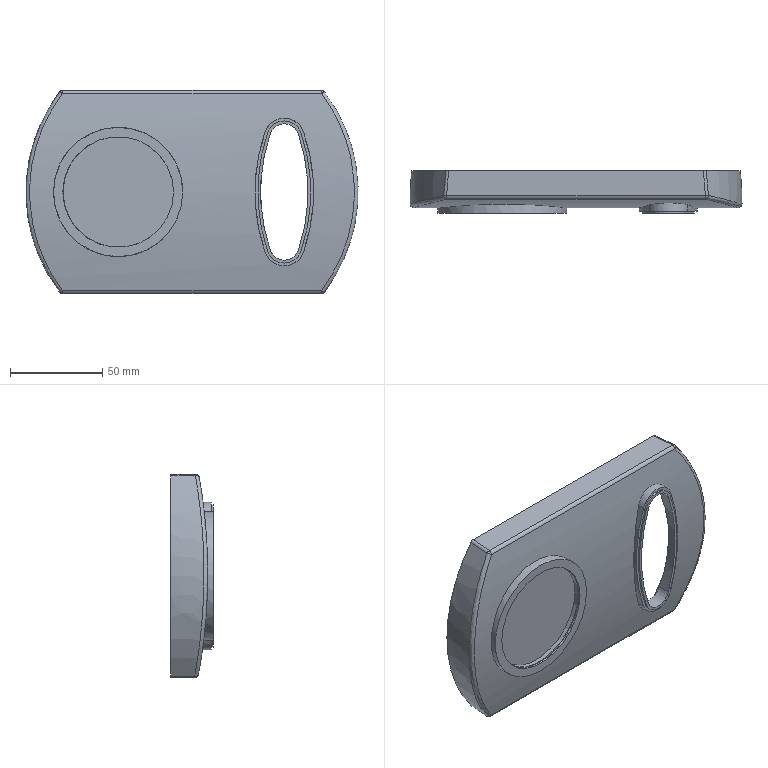Component | NX | UPPER_CASING | 1 solid | 78 faces | volume 58708 mm3 | plane 25 | cylinder 24 | spline 16 | sphere 8 | cone 5 | commonest cylinder face diameters 4 x4 194 x2 22 x2 200 x2 60 x2 16 x2 197 x2 19 x2